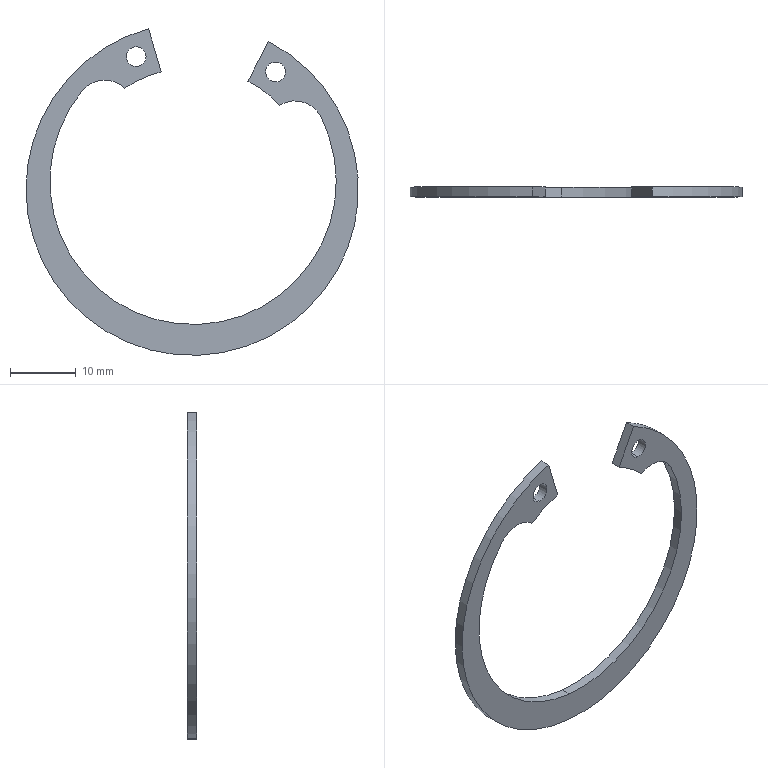Component | SolidWorks | 14-1 | 1 solid | 16 faces | box 50.5 x 1.5 x 49.61 mm | volume 798 mm3 | cylinder 12 | plane 4 | commonest cylinder face diameters 3 x4 50.5 x2 43.5 x2 36.9 x2 8.8 x2
STEP:
#1=CARTESIAN_POINT('',(0.487,-0.07087,0.5954));
#2=VERTEX_POINT('',#1);
#3=CARTESIAN_POINT('',(0.4998,-0.07087,0.7128));
#4=VERTEX_POINT('',#3);
#5=CARTESIAN_POINT('',(0.4934,-0.07087,0.6541));
#6=DIRECTION('',(0.,1.,0.));
#7=DIRECTION('',(-0.1087,0.,-0.9941));
#8=AXIS2_PLACEMENT_3D('',#5,#6,#7);
#9=CIRCLE('',#8,0.05906);
#10=EDGE_CURVE('',#2,#4,#9,.T.);
#11=ORIENTED_EDGE('',*,*,#10,.T.);
#12=CARTESIAN_POINT('',(0.4998,-0.1299,0.7128));
#13=VERTEX_POINT('',#12);
#14=CARTESIAN_POINT('',(0.4998,-0.07087,0.7128));
#15=DIRECTION('',(0.,-1.,0.));
#16=VECTOR('',#15,39.37);
#17=LINE('',#14,#16);
#18=EDGE_CURVE('',#4,#13,#17,.T.);
#19=ORIENTED_EDGE('',*,*,#18,.T.);
#20=CARTESIAN_POINT('',(0.487,-0.1299,0.5954));
#21=VERTEX_POINT('',#20);
#22=CARTESIAN_POINT('',(0.4934,-0.1299,0.6541));
#23=DIRECTION('',(0.,1.,0.));
#24=DIRECTION('',(-0.1087,0.,-0.9941));
#25=AXIS2_PLACEMENT_3D('',#22,#23,#24);
#26=CIRCLE('',#25,0.05906);
#27=EDGE_CURVE('',#21,#13,#26,.T.);
#28=ORIENTED_EDGE('',*,*,#27,.F.);
#29=CARTESIAN_POINT('',(0.487,-0.07087,0.5954));
#30=DIRECTION('',(0.,-1.,0.));
#31=VECTOR('',#30,39.37);
#32=LINE('',#29,#31);
#33=EDGE_CURVE('',#2,#21,#32,.T.);
#34=ORIENTED_EDGE('',*,*,#33,.F.);
#35=EDGE_LOOP('',(#11,#19,#28,#34));
#36=FACE_OUTER_BOUND('',#35,.T.);
#37=CARTESIAN_POINT('',(0.4934,-0.07087,0.6541));
#38=DIRECTION('',(0.,-1.,0.));
#39=DIRECTION('',(-0.1087,0.,-0.9941));
#40=AXIS2_PLACEMENT_3D('',#37,#38,#39);
#41=CYLINDRICAL_SURFACE('',#40,0.05906);
#42=ADVANCED_FACE('',(#36),#41,.F.);
#43=CARTESIAN_POINT('',(-0.3468,-0.07087,0.6865));
#44=VERTEX_POINT('',#43);
#45=CARTESIAN_POINT('',(-0.334,-0.07087,0.804));
#46=VERTEX_POINT('',#45);
#47=CARTESIAN_POINT('',(-0.3404,-0.07087,0.7453));
#48=DIRECTION('',(0.,1.,0.));
#49=DIRECTION('',(0.1087,0.,0.9941));
#50=AXIS2_PLACEMENT_3D('',#47,#48,#49);
#51=CIRCLE('',#50,0.05906);
#52=EDGE_CURVE('',#44,#46,#51,.T.);
#53=ORIENTED_EDGE('',*,*,#52,.T.);
#54=CARTESIAN_POINT('',(-0.334,-0.1299,0.804));
#55=VERTEX_POINT('',#54);
#56=CARTESIAN_POINT('',(-0.334,-0.07087,0.804));
#57=DIRECTION('',(0.,-1.,0.));
#58=VECTOR('',#57,39.37);
#59=LINE('',#56,#58);
#60=EDGE_CURVE('',#46,#55,#59,.T.);
#61=ORIENTED_EDGE('',*,*,#60,.T.);
#62=CARTESIAN_POINT('',(-0.3468,-0.1299,0.6865));
#63=VERTEX_POINT('',#62);
#64=CARTESIAN_POINT('',(-0.3404,-0.1299,0.7453));
#65=DIRECTION('',(0.,1.,0.));
#66=DIRECTION('',(0.1087,0.,0.9941));
#67=AXIS2_PLACEMENT_3D('',#64,#65,#66);
#68=CIRCLE('',#67,0.05906);
#69=EDGE_CURVE('',#63,#55,#68,.T.);
#70=ORIENTED_EDGE('',*,*,#69,.F.);
#71=CARTESIAN_POINT('',(-0.3468,-0.07087,0.6865));
#72=DIRECTION('',(0.,-1.,0.));
#73=VECTOR('',#72,39.37);
#74=LINE('',#71,#73);
#75=EDGE_CURVE('',#44,#63,#74,.T.);
#76=ORIENTED_EDGE('',*,*,#75,.F.);
#77=EDGE_LOOP('',(#53,#61,#70,#76));
#78=FACE_OUTER_BOUND('',#77,.T.);
#79=CARTESIAN_POINT('',(-0.3404,-0.07087,0.7453));
#80=DIRECTION('',(0.,-1.,0.));
#81=DIRECTION('',(-0.1087,0.,-0.9941));
#82=AXIS2_PLACEMENT_3D('',#79,#80,#81);
#83=CYLINDRICAL_SURFACE('',#82,0.05906);
#84=ADVANCED_FACE('',(#78),#83,.F.);
#85=CARTESIAN_POINT('',(-0.1132,-0.07087,-1.035));
#86=VERTEX_POINT('',#85);
#87=CARTESIAN_POINT('',(-0.2661,-0.07087,0.9123));
#88=VERTEX_POINT('',#87);
#89=CARTESIAN_POINT('',(-0.005135,-0.07087,-0.04696));
#90=DIRECTION('',(0.,1.,0.));
#91=DIRECTION('',(0.1087,0.,0.9941));
#92=AXIS2_PLACEMENT_3D('',#89,#90,#91);
#93=CIRCLE('',#92,0.9941);
#94=EDGE_CURVE('',#86,#88,#93,.T.);
#95=ORIENTED_EDGE('',*,*,#94,.F.);
#96=CARTESIAN_POINT('',(-0.1132,-0.1299,-1.035));
#97=VERTEX_POINT('',#96);
#98=CARTESIAN_POINT('',(-0.1132,-0.07087,-1.035));
#99=DIRECTION('',(0.,-1.,0.));
#100=VECTOR('',#99,39.37);
#101=LINE('',#98,#100);
#102=EDGE_CURVE('',#86,#97,#101,.T.);
#103=ORIENTED_EDGE('',*,*,#102,.T.);
#104=CARTESIAN_POINT('',(-0.2661,-0.1299,0.9123));
#105=VERTEX_POINT('',#104);
#106=CARTESIAN_POINT('',(-0.005135,-0.1299,-0.04696));
#107=DIRECTION('',(0.,1.,0.));
#108=DIRECTION('',(0.1087,0.,0.9941));
#109=AXIS2_PLACEMENT_3D('',#106,#107,#108);
#110=CIRCLE('',#109,0.9941);
#111=EDGE_CURVE('',#97,#105,#110,.T.);
#112=ORIENTED_EDGE('',*,*,#111,.T.);
#113=CARTESIAN_POINT('',(-0.2661,-0.07087,0.9123));
#114=DIRECTION('',(0.,-1.,0.));
#115=VECTOR('',#114,39.37);
#116=LINE('',#113,#115);
#117=EDGE_CURVE('',#88,#105,#116,.T.);
#118=ORIENTED_EDGE('',*,*,#117,.F.);
#119=EDGE_LOOP('',(#95,#103,#112,#118));
#120=FACE_OUTER_BOUND('',#119,.T.);
#121=CARTESIAN_POINT('',(-0.005135,-0.07087,-0.04696));
#122=DIRECTION('',(0.,-1.,0.));
#123=DIRECTION('',(-0.1087,0.,-0.9941));
#124=AXIS2_PLACEMENT_3D('',#121,#122,#123);
#125=CYLINDRICAL_SURFACE('',#124,0.9941);
#126=ADVANCED_FACE('',(#120),#125,.T.);
#127=CARTESIAN_POINT('',(-0.09307,-0.07087,-0.8512));
#128=VERTEX_POINT('',#127);
#129=CARTESIAN_POINT('',(0.7644,-0.07087,0.386));
#130=VERTEX_POINT('',#129);
#131=CARTESIAN_POINT('',(0.,-0.07087,0.));
#132=DIRECTION('',(0.,-1.,0.));
#133=DIRECTION('',(0.1087,0.,0.9941));
#134=AXIS2_PLACEMENT_3D('',#131,#132,#133);
#135=CIRCLE('',#134,0.8563);
#136=EDGE_CURVE('',#128,#130,#135,.T.);
#137=ORIENTED_EDGE('',*,*,#136,.F.);
#138=CARTESIAN_POINT('',(-0.09307,-0.1299,-0.8512));
#139=VERTEX_POINT('',#138);
#140=CARTESIAN_POINT('',(-0.09307,-0.07087,-0.8512));
#141=DIRECTION('',(0.,-1.,0.));
#142=VECTOR('',#141,39.37);
#143=LINE('',#140,#142);
#144=EDGE_CURVE('',#128,#139,#143,.T.);
#145=ORIENTED_EDGE('',*,*,#144,.T.);
#146=CARTESIAN_POINT('',(0.7644,-0.1299,0.386));
#147=VERTEX_POINT('',#146);
#148=CARTESIAN_POINT('',(0.,-0.1299,0.));
#149=DIRECTION('',(0.,-1.,0.));
#150=DIRECTION('',(0.1087,0.,0.9941));
#151=AXIS2_PLACEMENT_3D('',#148,#149,#150);
#152=CIRCLE('',#151,0.8563);
#153=EDGE_CURVE('',#139,#147,#152,.T.);
#154=ORIENTED_EDGE('',*,*,#153,.T.);
#155=CARTESIAN_POINT('',(0.7644,-0.07087,0.386));
#156=DIRECTION('',(0.,1.,0.));
#157=VECTOR('',#156,39.37);
#158=LINE('',#155,#157);
#159=EDGE_CURVE('',#147,#130,#158,.T.);
#160=ORIENTED_EDGE('',*,*,#159,.T.);
#161=EDGE_LOOP('',(#137,#145,#154,#160));
#162=FACE_OUTER_BOUND('',#161,.T.);
#163=CARTESIAN_POINT('',(0.,-0.07087,0.));
#164=DIRECTION('',(0.,-1.,0.));
#165=DIRECTION('',(-0.1087,0.,-0.9941));
#166=AXIS2_PLACEMENT_3D('',#163,#164,#165);
#167=CYLINDRICAL_SURFACE('',#166,0.8563);
#168=ADVANCED_FACE('',(#162),#167,.F.);
#169=ORIENTED_EDGE('',*,*,#52,.F.);
#170=CARTESIAN_POINT('',(-0.3404,-0.07087,0.7453));
#171=DIRECTION('',(0.,1.,0.));
#172=DIRECTION('',(0.1087,0.,0.9941));
#173=AXIS2_PLACEMENT_3D('',#170,#171,#172);
#174=CIRCLE('',#173,0.05906);
#175=EDGE_CURVE('',#46,#44,#174,.T.);
#176=ORIENTED_EDGE('',*,*,#175,.F.);
#177=EDGE_LOOP('',(#169,#176));
#178=FACE_BOUND('',#177,.T.);
#179=CARTESIAN_POINT('',(-0.1911,-0.07087,0.6552));
#180=VERTEX_POINT('',#179);
#181=CARTESIAN_POINT('',(-0.4085,-0.07087,0.5571));
#182=VERTEX_POINT('',#181);
#183=CARTESIAN_POINT('',(-0.005135,-0.07087,-0.04696));
#184=DIRECTION('',(0.,-1.,0.));
#185=DIRECTION('',(0.1087,0.,0.9941));
#186=AXIS2_PLACEMENT_3D('',#183,#184,#185);
#187=CIRCLE('',#186,0.7264);
#188=EDGE_CURVE('',#180,#182,#187,.T.);
#189=ORIENTED_EDGE('',*,*,#188,.T.);
#190=CARTESIAN_POINT('',(-0.6629,-0.07087,0.5421));
#191=VERTEX_POINT('',#190);
#192=CARTESIAN_POINT('',(-0.5288,-0.07087,0.4324));
#193=DIRECTION('',(0.,-1.,0.));
#194=DIRECTION('',(0.1087,0.,0.9941));
#195=AXIS2_PLACEMENT_3D('',#192,#193,#194);
#196=CIRCLE('',#195,0.1732);
#197=EDGE_CURVE('',#182,#191,#196,.T.);
#198=ORIENTED_EDGE('',*,*,#197,.T.);
#199=CARTESIAN_POINT('',(0.,-0.07087,0.));
#200=DIRECTION('',(0.,-1.,0.));
#201=DIRECTION('',(0.1087,0.,0.9941));
#202=AXIS2_PLACEMENT_3D('',#199,#200,#201);
#203=CIRCLE('',#202,0.8563);
#204=EDGE_CURVE('',#191,#128,#203,.T.);
#205=ORIENTED_EDGE('',*,*,#204,.T.);
#206=ORIENTED_EDGE('',*,*,#136,.T.);
#207=CARTESIAN_POINT('',(0.5193,-0.07087,0.4556));
#208=VERTEX_POINT('',#207);
#209=CARTESIAN_POINT('',(0.6097,-0.07087,0.3079));
#210=DIRECTION('',(0.,-1.,0.));
#211=DIRECTION('',(0.1087,0.,0.9941));
#212=AXIS2_PLACEMENT_3D('',#209,#210,#211);
#213=CIRCLE('',#212,0.1732);
#214=EDGE_CURVE('',#130,#208,#213,.T.);
#215=ORIENTED_EDGE('',*,*,#214,.T.);
#216=CARTESIAN_POINT('',(0.3282,-0.07087,0.5984));
#217=VERTEX_POINT('',#216);
#218=CARTESIAN_POINT('',(-0.005135,-0.07087,-0.04696));
#219=DIRECTION('',(0.,-1.,0.));
#220=DIRECTION('',(-0.1087,0.,-0.9941));
#221=AXIS2_PLACEMENT_3D('',#218,#219,#220);
#222=CIRCLE('',#221,0.7264);
#223=EDGE_CURVE('',#208,#217,#222,.T.);
#224=ORIENTED_EDGE('',*,*,#223,.T.);
#225=CARTESIAN_POINT('',(0.451,-0.07087,0.8363));
#226=VERTEX_POINT('',#225);
#227=CARTESIAN_POINT('',(0.3282,-0.07087,0.5984));
#228=DIRECTION('',(0.4589,0.,0.8885));
#229=VECTOR('',#228,39.37);
#230=LINE('',#227,#229);
#231=EDGE_CURVE('',#217,#226,#230,.T.);
#232=ORIENTED_EDGE('',*,*,#231,.T.);
#233=CARTESIAN_POINT('',(-0.005135,-0.07087,-0.04696));
#234=DIRECTION('',(0.,1.,0.));
#235=DIRECTION('',(0.1087,0.,0.9941));
#236=AXIS2_PLACEMENT_3D('',#233,#234,#235);
#237=CIRCLE('',#236,0.9941);
#238=EDGE_CURVE('',#226,#86,#237,.T.);
#239=ORIENTED_EDGE('',*,*,#238,.T.);
#240=ORIENTED_EDGE('',*,*,#94,.T.);
#241=CARTESIAN_POINT('',(-0.1911,-0.07087,0.6552));
#242=DIRECTION('',(0.28,0.,-0.96));
#243=VECTOR('',#242,39.37);
#244=LINE('',#241,#243);
#245=EDGE_CURVE('',#88,#180,#244,.T.);
#246=ORIENTED_EDGE('',*,*,#245,.T.);
#247=EDGE_LOOP('',(#189,#198,#205,#206,#215,#224,#232,#239,#240,#246));
#248=FACE_OUTER_BOUND('',#247,.T.);
#249=ORIENTED_EDGE('',*,*,#10,.F.);
#250=CARTESIAN_POINT('',(0.4934,-0.07087,0.6541));
#251=DIRECTION('',(0.,1.,0.));
#252=DIRECTION('',(-0.1087,0.,-0.9941));
#253=AXIS2_PLACEMENT_3D('',#250,#251,#252);
#254=CIRCLE('',#253,0.05906);
#255=EDGE_CURVE('',#4,#2,#254,.T.);
#256=ORIENTED_EDGE('',*,*,#255,.F.);
#257=EDGE_LOOP('',(#249,#256));
#258=FACE_BOUND('',#257,.T.);
#259=CARTESIAN_POINT('',(0.,-0.07087,0.));
#260=DIRECTION('',(0.,1.,0.));
#261=DIRECTION('',(0.1087,0.,0.9941));
#262=AXIS2_PLACEMENT_3D('',#259,#260,#261);
#263=PLANE('',#262);
#264=ADVANCED_FACE('',(#178,#248,#258),#263,.T.);
#265=CARTESIAN_POINT('',(-0.6629,-0.1299,0.5421));
#266=VERTEX_POINT('',#265);
#267=CARTESIAN_POINT('',(0.,-0.1299,0.));
#268=DIRECTION('',(0.,-1.,0.));
#269=DIRECTION('',(0.1087,0.,0.9941));
#270=AXIS2_PLACEMENT_3D('',#267,#268,#269);
#271=CIRCLE('',#270,0.8563);
#272=EDGE_CURVE('',#266,#139,#271,.T.);
#273=ORIENTED_EDGE('',*,*,#272,.F.);
#274=CARTESIAN_POINT('',(-0.4085,-0.1299,0.5571));
#275=VERTEX_POINT('',#274);
#276=CARTESIAN_POINT('',(-0.5288,-0.1299,0.4324));
#277=DIRECTION('',(0.,1.,0.));
#278=DIRECTION('',(0.1087,0.,0.9941));
#279=AXIS2_PLACEMENT_3D('',#276,#277,#278);
#280=CIRCLE('',#279,0.1732);
#281=EDGE_CURVE('',#266,#275,#280,.T.);
#282=ORIENTED_EDGE('',*,*,#281,.T.);
#283=CARTESIAN_POINT('',(-0.1911,-0.1299,0.6552));
#284=VERTEX_POINT('',#283);
#285=CARTESIAN_POINT('',(-0.005135,-0.1299,-0.04696));
#286=DIRECTION('',(0.,-1.,0.));
#287=DIRECTION('',(0.1087,0.,0.9941));
#288=AXIS2_PLACEMENT_3D('',#285,#286,#287);
#289=CIRCLE('',#288,0.7264);
#290=EDGE_CURVE('',#284,#275,#289,.T.);
#291=ORIENTED_EDGE('',*,*,#290,.F.);
#292=CARTESIAN_POINT('',(-0.1911,-0.1299,0.6552));
#293=DIRECTION('',(0.28,0.,-0.96));
#294=VECTOR('',#293,39.37);
#295=LINE('',#292,#294);
#296=EDGE_CURVE('',#105,#284,#295,.T.);
#297=ORIENTED_EDGE('',*,*,#296,.F.);
#298=ORIENTED_EDGE('',*,*,#111,.F.);
#299=CARTESIAN_POINT('',(0.451,-0.1299,0.8363));
#300=VERTEX_POINT('',#299);
#301=CARTESIAN_POINT('',(-0.005135,-0.1299,-0.04696));
#302=DIRECTION('',(0.,1.,0.));
#303=DIRECTION('',(0.1087,0.,0.9941));
#304=AXIS2_PLACEMENT_3D('',#301,#302,#303);
#305=CIRCLE('',#304,0.9941);
#306=EDGE_CURVE('',#300,#97,#305,.T.);
#307=ORIENTED_EDGE('',*,*,#306,.F.);
#308=CARTESIAN_POINT('',(0.3282,-0.1299,0.5984));
#309=VERTEX_POINT('',#308);
#310=CARTESIAN_POINT('',(0.3282,-0.1299,0.5984));
#311=DIRECTION('',(0.4589,0.,0.8885));
#312=VECTOR('',#311,39.37);
#313=LINE('',#310,#312);
#314=EDGE_CURVE('',#309,#300,#313,.T.);
#315=ORIENTED_EDGE('',*,*,#314,.F.);
#316=CARTESIAN_POINT('',(0.5193,-0.1299,0.4556));
#317=VERTEX_POINT('',#316);
#318=CARTESIAN_POINT('',(-0.005135,-0.1299,-0.04696));
#319=DIRECTION('',(0.,-1.,0.));
#320=DIRECTION('',(-0.1087,0.,-0.9941));
#321=AXIS2_PLACEMENT_3D('',#318,#319,#320);
#322=CIRCLE('',#321,0.7264);
#323=EDGE_CURVE('',#317,#309,#322,.T.);
#324=ORIENTED_EDGE('',*,*,#323,.F.);
#325=CARTESIAN_POINT('',(0.6097,-0.1299,0.3079));
#326=DIRECTION('',(0.,1.,0.));
#327=DIRECTION('',(0.1087,0.,0.9941));
#328=AXIS2_PLACEMENT_3D('',#325,#326,#327);
#329=CIRCLE('',#328,0.1732);
#330=EDGE_CURVE('',#317,#147,#329,.T.);
#331=ORIENTED_EDGE('',*,*,#330,.T.);
#332=ORIENTED_EDGE('',*,*,#153,.F.);
#333=EDGE_LOOP('',(#273,#282,#291,#297,#298,#307,#315,#324,#331,#332));
#334=FACE_OUTER_BOUND('',#333,.T.);
#335=ORIENTED_EDGE('',*,*,#69,.T.);
#336=CARTESIAN_POINT('',(-0.3404,-0.1299,0.7453));
#337=DIRECTION('',(0.,1.,0.));
#338=DIRECTION('',(0.1087,0.,0.9941));
#339=AXIS2_PLACEMENT_3D('',#336,#337,#338);
#340=CIRCLE('',#339,0.05906);
#341=EDGE_CURVE('',#55,#63,#340,.T.);
#342=ORIENTED_EDGE('',*,*,#341,.T.);
#343=EDGE_LOOP('',(#335,#342));
#344=FACE_BOUND('',#343,.T.);
#345=ORIENTED_EDGE('',*,*,#27,.T.);
#346=CARTESIAN_POINT('',(0.4934,-0.1299,0.6541));
#347=DIRECTION('',(0.,1.,0.));
#348=DIRECTION('',(-0.1087,0.,-0.9941));
#349=AXIS2_PLACEMENT_3D('',#346,#347,#348);
#350=CIRCLE('',#349,0.05906);
#351=EDGE_CURVE('',#13,#21,#350,.T.);
#352=ORIENTED_EDGE('',*,*,#351,.T.);
#353=EDGE_LOOP('',(#345,#352));
#354=FACE_BOUND('',#353,.T.);
#355=CARTESIAN_POINT('',(0.,-0.1299,0.));
#356=DIRECTION('',(0.,1.,0.));
#357=DIRECTION('',(0.1087,0.,0.9941));
#358=AXIS2_PLACEMENT_3D('',#355,#356,#357);
#359=PLANE('',#358);
#360=ADVANCED_FACE('',(#334,#344,#354),#359,.F.);
#361=ORIENTED_EDGE('',*,*,#144,.F.);
#362=ORIENTED_EDGE('',*,*,#204,.F.);
#363=CARTESIAN_POINT('',(-0.6629,-0.07087,0.5421));
#364=DIRECTION('',(0.,-1.,0.));
#365=VECTOR('',#364,39.37);
#366=LINE('',#363,#365);
#367=EDGE_CURVE('',#191,#266,#366,.T.);
#368=ORIENTED_EDGE('',*,*,#367,.T.);
#369=ORIENTED_EDGE('',*,*,#272,.T.);
#370=EDGE_LOOP('',(#361,#362,#368,#369));
#371=FACE_OUTER_BOUND('',#370,.T.);
#372=CARTESIAN_POINT('',(0.,-0.07087,0.));
#373=DIRECTION('',(0.,-1.,0.));
#374=DIRECTION('',(-0.1087,0.,-0.9941));
#375=AXIS2_PLACEMENT_3D('',#372,#373,#374);
#376=CYLINDRICAL_SURFACE('',#375,0.8563);
#377=ADVANCED_FACE('',(#371),#376,.F.);
#378=ORIENTED_EDGE('',*,*,#323,.T.);
#379=CARTESIAN_POINT('',(0.3282,-0.07087,0.5984));
#380=DIRECTION('',(0.,-1.,0.));
#381=VECTOR('',#380,39.37);
#382=LINE('',#379,#381);
#383=EDGE_CURVE('',#217,#309,#382,.T.);
#384=ORIENTED_EDGE('',*,*,#383,.F.);
#385=ORIENTED_EDGE('',*,*,#223,.F.);
#386=CARTESIAN_POINT('',(0.5193,-0.07087,0.4556));
#387=DIRECTION('',(0.,-1.,0.));
#388=VECTOR('',#387,39.37);
#389=LINE('',#386,#388);
#390=EDGE_CURVE('',#208,#317,#389,.T.);
#391=ORIENTED_EDGE('',*,*,#390,.T.);
#392=EDGE_LOOP('',(#378,#384,#385,#391));
#393=FACE_OUTER_BOUND('',#392,.T.);
#394=CARTESIAN_POINT('',(-0.005135,-0.07087,-0.04696));
#395=DIRECTION('',(0.,-1.,0.));
#396=DIRECTION('',(-0.1087,0.,-0.9941));
#397=AXIS2_PLACEMENT_3D('',#394,#395,#396);
#398=CYLINDRICAL_SURFACE('',#397,0.7264);
#399=ADVANCED_FACE('',(#393),#398,.F.);
#400=ORIENTED_EDGE('',*,*,#314,.T.);
#401=CARTESIAN_POINT('',(0.451,-0.07087,0.8363));
#402=DIRECTION('',(0.,-1.,0.));
#403=VECTOR('',#402,39.37);
#404=LINE('',#401,#403);
#405=EDGE_CURVE('',#226,#300,#404,.T.);
#406=ORIENTED_EDGE('',*,*,#405,.F.);
#407=ORIENTED_EDGE('',*,*,#231,.F.);
#408=ORIENTED_EDGE('',*,*,#383,.T.);
#409=EDGE_LOOP('',(#400,#406,#407,#408));
#410=FACE_OUTER_BOUND('',#409,.T.);
#411=CARTESIAN_POINT('',(0.3282,-0.07087,0.5984));
#412=DIRECTION('',(0.8885,0.,-0.4589));
#413=DIRECTION('',(-0.4589,0.,-0.8885));
#414=AXIS2_PLACEMENT_3D('',#411,#412,#413);
#415=PLANE('',#414);
#416=ADVANCED_FACE('',(#410),#415,.F.);
#417=ORIENTED_EDGE('',*,*,#102,.F.);
#418=ORIENTED_EDGE('',*,*,#238,.F.);
#419=ORIENTED_EDGE('',*,*,#405,.T.);
#420=ORIENTED_EDGE('',*,*,#306,.T.);
#421=EDGE_LOOP('',(#417,#418,#419,#420));
#422=FACE_OUTER_BOUND('',#421,.T.);
#423=CARTESIAN_POINT('',(-0.005135,-0.07087,-0.04696));
#424=DIRECTION('',(0.,-1.,0.));
#425=DIRECTION('',(-0.1087,0.,-0.9941));
#426=AXIS2_PLACEMENT_3D('',#423,#424,#425);
#427=CYLINDRICAL_SURFACE('',#426,0.9941);
#428=ADVANCED_FACE('',(#422),#427,.T.);
#429=ORIENTED_EDGE('',*,*,#296,.T.);
#430=CARTESIAN_POINT('',(-0.1911,-0.07087,0.6552));
#431=DIRECTION('',(0.,-1.,0.));
#432=VECTOR('',#431,39.37);
#433=LINE('',#430,#432);
#434=EDGE_CURVE('',#180,#284,#433,.T.);
#435=ORIENTED_EDGE('',*,*,#434,.F.);
#436=ORIENTED_EDGE('',*,*,#245,.F.);
#437=ORIENTED_EDGE('',*,*,#117,.T.);
#438=EDGE_LOOP('',(#429,#435,#436,#437));
#439=FACE_OUTER_BOUND('',#438,.T.);
#440=CARTESIAN_POINT('',(-0.1911,-0.07087,0.6552));
#441=DIRECTION('',(-0.96,0.,-0.28));
#442=DIRECTION('',(-0.28,0.,0.96));
#443=AXIS2_PLACEMENT_3D('',#440,#441,#442);
#444=PLANE('',#443);
#445=ADVANCED_FACE('',(#439),#444,.F.);
#446=ORIENTED_EDGE('',*,*,#290,.T.);
#447=CARTESIAN_POINT('',(-0.4085,-0.07087,0.5571));
#448=DIRECTION('',(0.,-1.,0.));
#449=VECTOR('',#448,39.37);
#450=LINE('',#447,#449);
#451=EDGE_CURVE('',#182,#275,#450,.T.);
#452=ORIENTED_EDGE('',*,*,#451,.F.);
#453=ORIENTED_EDGE('',*,*,#188,.F.);
#454=ORIENTED_EDGE('',*,*,#434,.T.);
#455=EDGE_LOOP('',(#446,#452,#453,#454));
#456=FACE_OUTER_BOUND('',#455,.T.);
#457=CARTESIAN_POINT('',(-0.005135,-0.07087,-0.04696));
#458=DIRECTION('',(0.,-1.,0.));
#459=DIRECTION('',(-0.1087,0.,-0.9941));
#460=AXIS2_PLACEMENT_3D('',#457,#458,#459);
#461=CYLINDRICAL_SURFACE('',#460,0.7264);
#462=ADVANCED_FACE('',(#456),#461,.F.);
#463=ORIENTED_EDGE('',*,*,#60,.F.);
#464=ORIENTED_EDGE('',*,*,#175,.T.);
#465=ORIENTED_EDGE('',*,*,#75,.T.);
#466=ORIENTED_EDGE('',*,*,#341,.F.);
#467=EDGE_LOOP('',(#463,#464,#465,#466));
#468=FACE_OUTER_BOUND('',#467,.T.);
#469=CARTESIAN_POINT('',(-0.3404,-0.07087,0.7453));
#470=DIRECTION('',(0.,-1.,0.));
#471=DIRECTION('',(-0.1087,0.,-0.9941));
#472=AXIS2_PLACEMENT_3D('',#469,#470,#471);
#473=CYLINDRICAL_SURFACE('',#472,0.05906);
#474=ADVANCED_FACE('',(#468),#473,.F.);
#475=ORIENTED_EDGE('',*,*,#18,.F.);
#476=ORIENTED_EDGE('',*,*,#255,.T.);
#477=ORIENTED_EDGE('',*,*,#33,.T.);
#478=ORIENTED_EDGE('',*,*,#351,.F.);
#479=EDGE_LOOP('',(#475,#476,#477,#478));
#480=FACE_OUTER_BOUND('',#479,.T.);
#481=CARTESIAN_POINT('',(0.4934,-0.07087,0.6541));
#482=DIRECTION('',(0.,-1.,0.));
#483=DIRECTION('',(-0.1087,0.,-0.9941));
#484=AXIS2_PLACEMENT_3D('',#481,#482,#483);
#485=CYLINDRICAL_SURFACE('',#484,0.05906);
#486=ADVANCED_FACE('',(#480),#485,.F.);
#487=ORIENTED_EDGE('',*,*,#214,.F.);
#488=ORIENTED_EDGE('',*,*,#159,.F.);
#489=ORIENTED_EDGE('',*,*,#330,.F.);
#490=ORIENTED_EDGE('',*,*,#390,.F.);
#491=EDGE_LOOP('',(#487,#488,#489,#490));
#492=FACE_OUTER_BOUND('',#491,.T.);
#493=CARTESIAN_POINT('',(0.6097,-0.07087,0.3079));
#494=DIRECTION('',(0.,-1.,0.));
#495=DIRECTION('',(-0.1087,0.,-0.9941));
#496=AXIS2_PLACEMENT_3D('',#493,#494,#495);
#497=CYLINDRICAL_SURFACE('',#496,0.1732);
#498=ADVANCED_FACE('',(#492),#497,.F.);
#499=ORIENTED_EDGE('',*,*,#197,.F.);
#500=ORIENTED_EDGE('',*,*,#451,.T.);
#501=ORIENTED_EDGE('',*,*,#281,.F.);
#502=ORIENTED_EDGE('',*,*,#367,.F.);
#503=EDGE_LOOP('',(#499,#500,#501,#502));
#504=FACE_OUTER_BOUND('',#503,.T.);
#505=CARTESIAN_POINT('',(-0.5288,-0.07087,0.4324));
#506=DIRECTION('',(0.,-1.,0.));
#507=DIRECTION('',(-0.1087,0.,-0.9941));
#508=AXIS2_PLACEMENT_3D('',#505,#506,#507);
#509=CYLINDRICAL_SURFACE('',#508,0.1732);
#510=ADVANCED_FACE('',(#504),#509,.F.);
#511=CLOSED_SHELL('',(#42,#84,#126,#168,#264,#360,#377,#399,#416,#428,#445,#462,#474,#486,#498,#510));
#512=MANIFOLD_SOLID_BREP('',#511);
#513=CARTESIAN_POINT('',(0.,0.,0.));
#514=DIRECTION('',(0.,0.,1.));
#515=DIRECTION('',(1.,0.,0.));
#516=AXIS2_PLACEMENT_3D('',#513,#514,#515);
#517=(LENGTH_UNIT()NAMED_UNIT(*)SI_UNIT($,.METRE.));
#518=LENGTH_MEASURE_WITH_UNIT(LENGTH_MEASURE(0.0254),#517);
#519=DIMENSIONAL_EXPONENTS(1.,0.,0.,0.,0.,0.,0.);
#520=(CONVERSION_BASED_UNIT('',#518)LENGTH_UNIT()NAMED_UNIT(#519));
#521=UNCERTAINTY_MEASURE_WITH_UNIT(LENGTH_MEASURE(0.00001),#520,'','');
#522=(NAMED_UNIT(*)PLANE_ANGLE_UNIT()SI_UNIT($,.RADIAN.));
#523=(NAMED_UNIT(*)SI_UNIT($,.STERADIAN.)SOLID_ANGLE_UNIT());
#524=(GEOMETRIC_REPRESENTATION_CONTEXT(3)GLOBAL_UNCERTAINTY_ASSIGNED_CONTEXT((#521))GLOBAL_UNIT_ASSIGNED_CONTEXT((#520,#522,#523))REPRESENTATION_CONTEXT('',''));
#525=ADVANCED_BREP_SHAPE_REPRESENTATION('',(#512,#516),#524);
#526=COLOUR_RGB('',0.7922,0.8196,0.9333);
#527=FILL_AREA_STYLE_COLOUR('',#526);
#528=FILL_AREA_STYLE('',(#527));
#529=SURFACE_STYLE_FILL_AREA(#528);
#530=SURFACE_SIDE_STYLE('',(#529));
#531=SURFACE_STYLE_USAGE(.BOTH.,#530);
#532=PRESENTATION_STYLE_ASSIGNMENT((#531));
#533=STYLED_ITEM('',(#532),#512);
#534=PRESENTATION_LAYER_ASSIGNMENT('','',(#533));
#535=(LENGTH_UNIT()NAMED_UNIT(*)SI_UNIT($,.METRE.));
#536=LENGTH_MEASURE_WITH_UNIT(LENGTH_MEASURE(0.0254),#535);
#537=DIMENSIONAL_EXPONENTS(1.,0.,0.,0.,0.,0.,0.);
#538=(CONVERSION_BASED_UNIT('',#536)LENGTH_UNIT()NAMED_UNIT(#537));
#539=UNCERTAINTY_MEASURE_WITH_UNIT(LENGTH_MEASURE(0.00001),#538,'','');
#540=(NAMED_UNIT(*)PLANE_ANGLE_UNIT()SI_UNIT($,.RADIAN.));
#541=(NAMED_UNIT(*)SI_UNIT($,.STERADIAN.)SOLID_ANGLE_UNIT());
#542=(GEOMETRIC_REPRESENTATION_CONTEXT(3)GLOBAL_UNCERTAINTY_ASSIGNED_CONTEXT((#539))GLOBAL_UNIT_ASSIGNED_CONTEXT((#538,#540,#541))REPRESENTATION_CONTEXT('',''));
#543=MECHANICAL_DESIGN_GEOMETRIC_PRESENTATION_REPRESENTATION('',(#533),#542);